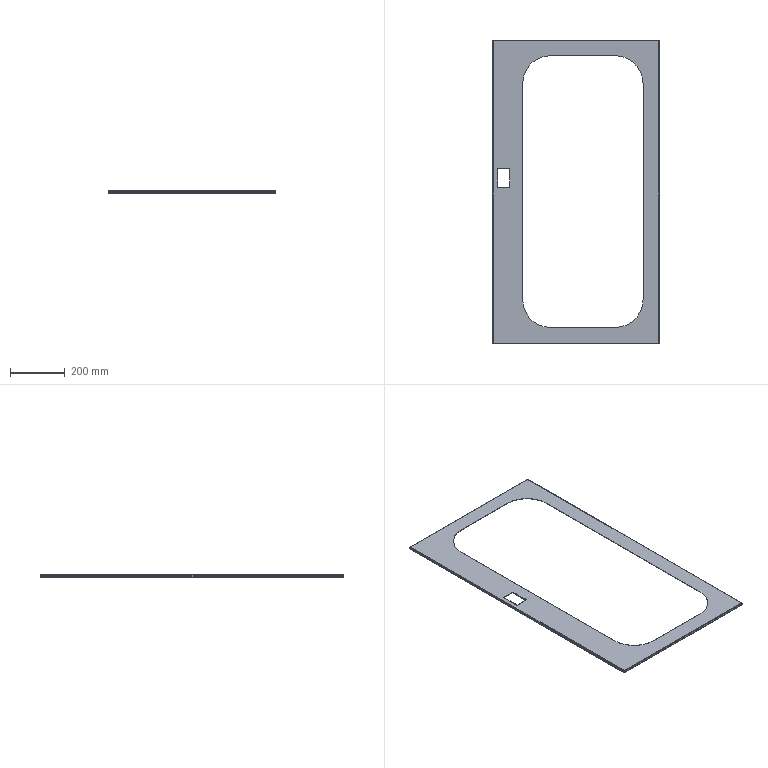Component | SolidWorks | UpperDoorFrame-1_UpperRearDoor-1 | 1 solid | 92 faces | volume 447059 mm3 | plane 56 | cylinder 20 | spline 16 | commonest cylinder face diameters 4.473 x8 1.473 x8 200 x4